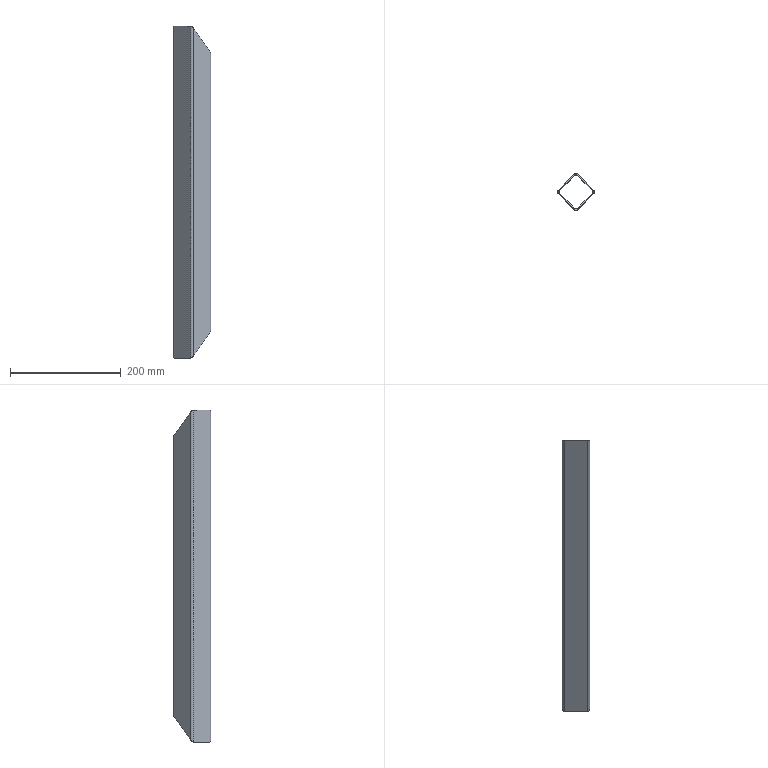Component | NX | SLID_FRAME_BEAM1_2 | 1 solid | 18 faces | volume 211200 mm3 | plane 10 | cylinder 8 | commonest cylinder face diameters 8 x8